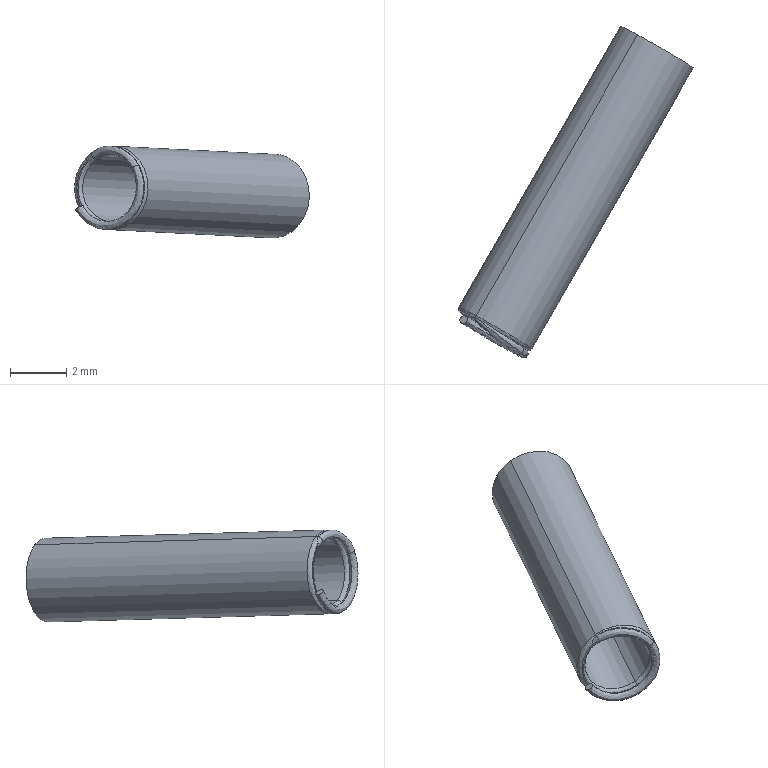Component | SolidWorks | ur3_15-0710z0-123-1 | 1 solid | 18 faces | box 8.38 x 11.84 x 3.29 mm | volume 30 mm3 | spline 11 | cylinder 4 | plane 3 | commonest cylinder face diameters 3 x2 2.4 x2
STEP:
#1=COLOUR_RGB('',0.7922,0.8196,0.9333);
#2=FILL_AREA_STYLE_COLOUR('',#1);
#3=FILL_AREA_STYLE('',(#2));
#4=SURFACE_STYLE_FILL_AREA(#3);
#5=SURFACE_SIDE_STYLE('',(#4));
#6=SURFACE_STYLE_USAGE(.BOTH.,#5);
#7=PRESENTATION_STYLE_ASSIGNMENT((#6));
#8=CARTESIAN_POINT('',(-3.463,-3.815,3.274));
#9=VERTEX_POINT('',#8);
#10=CARTESIAN_POINT('',(-3.409,-3.849,3.175));
#11=VERTEX_POINT('',#10);
#12=CARTESIAN_POINT('',(-3.436,-3.832,3.225));
#13=DIRECTION('',(0.4977,0.867,-0.02519));
#14=DIRECTION('',(-0.4585,0.2877,0.8408));
#15=AXIS2_PLACEMENT_3D('',#12,#13,#14);
#16=CIRCLE('',#15,0.05906);
#17=EDGE_CURVE('',#9,#11,#16,.T.);
#18=ORIENTED_EDGE('',*,*,#17,.F.);
#19=CARTESIAN_POINT('',(-3.464,-3.818,3.274));
#20=VERTEX_POINT('',#19);
#21=CARTESIAN_POINT('',(-3.461,-3.817,3.27));
#22=DIRECTION('',(0.7362,-0.4069,0.5407));
#23=DIRECTION('',(-0.4585,0.2877,0.8408));
#24=AXIS2_PLACEMENT_3D('',#21,#22,#23);
#25=CIRCLE('',#24,0.005906);
#26=EDGE_CURVE('',#9,#20,#25,.T.);
#27=ORIENTED_EDGE('',*,*,#26,.T.);
#28=CARTESIAN_POINT('',(-3.463,-3.819,3.275));
#29=VERTEX_POINT('',#28);
#30=CARTESIAN_POINT('',(-3.464,-3.818,3.274));
#31=CARTESIAN_POINT('',(-3.464,-3.819,3.274));
#32=CARTESIAN_POINT('',(-3.464,-3.819,3.274));
#33=CARTESIAN_POINT('',(-3.463,-3.819,3.275));
#34=B_SPLINE_CURVE_WITH_KNOTS('',3,(#30,#31,#32,#33),.UNSPECIFIED.,.F.,.F.,(4,4),(0.0003544,0.0003919),.UNSPECIFIED.);
#35=EDGE_CURVE('',#20,#29,#34,.T.);
#36=ORIENTED_EDGE('',*,*,#35,.T.);
#37=CARTESIAN_POINT('',(-3.461,-3.82,3.276));
#38=VERTEX_POINT('',#37);
#39=CARTESIAN_POINT('',(-3.463,-3.819,3.275));
#40=CARTESIAN_POINT('',(-3.463,-3.819,3.275));
#41=CARTESIAN_POINT('',(-3.462,-3.82,3.276));
#42=CARTESIAN_POINT('',(-3.461,-3.82,3.276));
#43=B_SPLINE_CURVE_WITH_KNOTS('',3,(#39,#40,#41,#42),.UNSPECIFIED.,.F.,.F.,(4,4),(0.0003919,0.0004641),.UNSPECIFIED.);
#44=EDGE_CURVE('',#29,#38,#43,.T.);
#45=ORIENTED_EDGE('',*,*,#44,.T.);
#46=CARTESIAN_POINT('',(-3.399,-3.86,3.255));
#47=VERTEX_POINT('',#46);
#48=CARTESIAN_POINT('',(-3.461,-3.82,3.276));
#49=CARTESIAN_POINT('',(-3.456,-3.823,3.28));
#50=CARTESIAN_POINT('',(-3.45,-3.826,3.282));
#51=CARTESIAN_POINT('',(-3.438,-3.834,3.283));
#52=CARTESIAN_POINT('',(-3.432,-3.838,3.282));
#53=CARTESIAN_POINT('',(-3.423,-3.844,3.279));
#54=CARTESIAN_POINT('',(-3.421,-3.845,3.278));
#55=CARTESIAN_POINT('',(-3.415,-3.849,3.275));
#56=CARTESIAN_POINT('',(-3.413,-3.85,3.273));
#57=CARTESIAN_POINT('',(-3.406,-3.855,3.266));
#58=CARTESIAN_POINT('',(-3.402,-3.858,3.261));
#59=CARTESIAN_POINT('',(-3.399,-3.86,3.255));
#60=B_SPLINE_CURVE_WITH_KNOTS('',3,(#48,#49,#50,#51,#52,#53,#54,#55,#56,#57,#58,#59),.UNSPECIFIED.,.F.,.F.,(4,2,2,2,2,4),(0.0004641,0.001005,0.001546,0.001817,0.002088,0.002629),.UNSPECIFIED.);
#61=EDGE_CURVE('',#38,#47,#60,.T.);
#62=ORIENTED_EDGE('',*,*,#61,.T.);
#63=CARTESIAN_POINT('',(-3.414,-3.853,3.179));
#64=VERTEX_POINT('',#63);
#65=CARTESIAN_POINT('',(-3.439,-3.837,3.225));
#66=DIRECTION('',(0.4977,0.867,-0.02519));
#67=DIRECTION('',(0.4585,-0.2877,-0.8408));
#68=AXIS2_PLACEMENT_3D('',#65,#66,#67);
#69=CIRCLE('',#68,0.05466);
#70=EDGE_CURVE('',#47,#64,#69,.T.);
#71=ORIENTED_EDGE('',*,*,#70,.T.);
#72=CARTESIAN_POINT('',(-3.412,-3.848,3.18));
#73=DIRECTION('',(-0.7362,0.4069,-0.5407));
#74=DIRECTION('',(0.4585,-0.2877,-0.8408));
#75=AXIS2_PLACEMENT_3D('',#72,#73,#74);
#76=CIRCLE('',#75,0.005906);
#77=EDGE_CURVE('',#11,#64,#76,.T.);
#78=ORIENTED_EDGE('',*,*,#77,.F.);
#79=EDGE_LOOP('',(#18,#27,#36,#45,#62,#71,#78));
#80=FACE_OUTER_BOUND('',#79,.T.);
#81=CARTESIAN_POINT('',(-3.463,-3.815,3.274));
#82=CARTESIAN_POINT('',(-3.376,-3.864,3.338));
#83=CARTESIAN_POINT('',(-3.322,-3.897,3.239));
#84=CARTESIAN_POINT('',(-3.409,-3.849,3.175));
#85=CARTESIAN_POINT('',(-3.465,-3.818,3.275));
#86=CARTESIAN_POINT('',(-3.378,-3.866,3.338));
#87=CARTESIAN_POINT('',(-3.324,-3.9,3.239));
#88=CARTESIAN_POINT('',(-3.411,-3.852,3.175));
#89=CARTESIAN_POINT('',(-3.465,-3.82,3.273));
#90=CARTESIAN_POINT('',(-3.381,-3.867,3.335));
#91=CARTESIAN_POINT('',(-3.328,-3.9,3.239));
#92=CARTESIAN_POINT('',(-3.412,-3.853,3.177));
#93=CARTESIAN_POINT('',(-3.464,-3.822,3.271));
#94=CARTESIAN_POINT('',(-3.384,-3.866,3.33));
#95=CARTESIAN_POINT('',(-3.334,-3.898,3.238));
#96=CARTESIAN_POINT('',(-3.414,-3.853,3.179));
#97=(BOUNDED_SURFACE()B_SPLINE_SURFACE(3,3,((#81,#82,#83,#84),(#85,#86,#87,#88),(#89,#90,#91,#92),(#93,#94,#95,#96)),.UNSPECIFIED.,.F.,.F.,.T.)B_SPLINE_SURFACE_WITH_KNOTS((4,4),(4,4),(0.,1.),(0.,1.),.UNSPECIFIED.)GEOMETRIC_REPRESENTATION_ITEM()RATIONAL_B_SPLINE_SURFACE(((1.,0.3333,0.3333,1.),(0.8617,0.2872,0.2872,0.8617),(0.8617,0.2872,0.2872,0.8617),(1.,0.3333,0.3333,1.)))REPRESENTATION_ITEM('')SURFACE());
#98=ADVANCED_FACE('',(#80),#97,.T.);
#99=CARTESIAN_POINT('',(-3.463,-3.822,3.27));
#100=VERTEX_POINT('',#99);
#101=CARTESIAN_POINT('',(-3.415,-3.852,3.18));
#102=VERTEX_POINT('',#101);
#103=CARTESIAN_POINT('',(-3.439,-3.837,3.225));
#104=DIRECTION('',(0.4977,0.867,-0.02519));
#105=DIRECTION('',(-0.4585,0.2877,0.8408));
#106=AXIS2_PLACEMENT_3D('',#103,#104,#105);
#107=CIRCLE('',#106,0.05315);
#108=EDGE_CURVE('',#100,#102,#107,.T.);
#109=ORIENTED_EDGE('',*,*,#108,.F.);
#110=CARTESIAN_POINT('',(-3.458,-3.818,3.265));
#111=VERTEX_POINT('',#110);
#112=CARTESIAN_POINT('',(-3.46,-3.817,3.27));
#113=DIRECTION('',(0.7362,-0.4069,0.5407));
#114=DIRECTION('',(-0.4585,0.2877,0.8408));
#115=AXIS2_PLACEMENT_3D('',#112,#113,#114);
#116=CIRCLE('',#115,0.005906);
#117=EDGE_CURVE('',#100,#111,#116,.T.);
#118=ORIENTED_EDGE('',*,*,#117,.T.);
#119=CARTESIAN_POINT('',(-3.414,-3.846,3.185));
#120=VERTEX_POINT('',#119);
#121=CARTESIAN_POINT('',(-3.436,-3.832,3.225));
#122=DIRECTION('',(0.4977,0.867,-0.02519));
#123=DIRECTION('',(0.4585,-0.2877,-0.8408));
#124=AXIS2_PLACEMENT_3D('',#121,#122,#123);
#125=CIRCLE('',#124,0.04724);
#126=EDGE_CURVE('',#111,#120,#125,.T.);
#127=ORIENTED_EDGE('',*,*,#126,.T.);
#128=CARTESIAN_POINT('',(-3.412,-3.847,3.18));
#129=DIRECTION('',(-0.7362,0.4069,-0.5407));
#130=DIRECTION('',(0.4585,-0.2877,-0.8408));
#131=AXIS2_PLACEMENT_3D('',#128,#129,#130);
#132=CIRCLE('',#131,0.005906);
#133=EDGE_CURVE('',#102,#120,#132,.T.);
#134=ORIENTED_EDGE('',*,*,#133,.F.);
#135=EDGE_LOOP('',(#109,#118,#127,#134));
#136=FACE_OUTER_BOUND('',#135,.T.);
#137=CARTESIAN_POINT('',(-3.463,-3.822,3.27));
#138=CARTESIAN_POINT('',(-3.385,-3.865,3.327));
#139=CARTESIAN_POINT('',(-3.336,-3.896,3.238));
#140=CARTESIAN_POINT('',(-3.415,-3.852,3.18));
#141=CARTESIAN_POINT('',(-3.462,-3.823,3.267));
#142=CARTESIAN_POINT('',(-3.389,-3.863,3.32));
#143=CARTESIAN_POINT('',(-3.343,-3.892,3.237));
#144=CARTESIAN_POINT('',(-3.416,-3.852,3.183));
#145=CARTESIAN_POINT('',(-3.459,-3.821,3.265));
#146=CARTESIAN_POINT('',(-3.39,-3.86,3.316));
#147=CARTESIAN_POINT('',(-3.347,-3.887,3.236));
#148=CARTESIAN_POINT('',(-3.416,-3.849,3.185));
#149=CARTESIAN_POINT('',(-3.458,-3.818,3.265));
#150=CARTESIAN_POINT('',(-3.388,-3.857,3.316));
#151=CARTESIAN_POINT('',(-3.345,-3.884,3.236));
#152=CARTESIAN_POINT('',(-3.414,-3.846,3.185));
#153=(BOUNDED_SURFACE()B_SPLINE_SURFACE(3,3,((#137,#138,#139,#140),(#141,#142,#143,#144),(#145,#146,#147,#148),(#149,#150,#151,#152)),.UNSPECIFIED.,.F.,.F.,.T.)B_SPLINE_SURFACE_WITH_KNOTS((4,4),(4,4),(0.,1.),(0.,1.),.UNSPECIFIED.)GEOMETRIC_REPRESENTATION_ITEM()RATIONAL_B_SPLINE_SURFACE(((1.,0.3333,0.3333,1.),(0.8047,0.2682,0.2682,0.8047),(0.8047,0.2682,0.2682,0.8047),(1.,0.3333,0.3333,1.)))REPRESENTATION_ITEM('')SURFACE());
#154=ADVANCED_FACE('',(#136),#153,.T.);
#155=ORIENTED_EDGE('',*,*,#108,.T.);
#156=CARTESIAN_POINT('',(-3.42,-3.856,3.185));
#157=VERTEX_POINT('',#156);
#158=CARTESIAN_POINT('',(-3.418,-3.858,3.18));
#159=DIRECTION('',(0.7362,-0.4069,0.5407));
#160=DIRECTION('',(0.4585,-0.2877,-0.8408));
#161=AXIS2_PLACEMENT_3D('',#158,#159,#160);
#162=CIRCLE('',#161,0.005906);
#163=EDGE_CURVE('',#102,#157,#162,.T.);
#164=ORIENTED_EDGE('',*,*,#163,.T.);
#165=CARTESIAN_POINT('',(-3.407,-3.862,3.251));
#166=VERTEX_POINT('',#165);
#167=CARTESIAN_POINT('',(-3.442,-3.842,3.225));
#168=DIRECTION('',(-0.4977,-0.867,0.02519));
#169=DIRECTION('',(-0.4585,0.2877,0.8408));
#170=AXIS2_PLACEMENT_3D('',#167,#168,#169);
#171=CIRCLE('',#170,0.04724);
#172=EDGE_CURVE('',#157,#166,#171,.T.);
#173=ORIENTED_EDGE('',*,*,#172,.T.);
#174=CARTESIAN_POINT('',(-3.462,-3.825,3.267));
#175=VERTEX_POINT('',#174);
#176=CARTESIAN_POINT('',(-3.462,-3.825,3.267));
#177=CARTESIAN_POINT('',(-3.458,-3.828,3.269));
#178=CARTESIAN_POINT('',(-3.453,-3.831,3.271));
#179=CARTESIAN_POINT('',(-3.445,-3.837,3.273));
#180=CARTESIAN_POINT('',(-3.442,-3.839,3.273));
#181=CARTESIAN_POINT('',(-3.437,-3.842,3.272));
#182=CARTESIAN_POINT('',(-3.436,-3.843,3.272));
#183=CARTESIAN_POINT('',(-3.434,-3.844,3.272));
#184=CARTESIAN_POINT('',(-3.432,-3.845,3.271));
#185=CARTESIAN_POINT('',(-3.431,-3.846,3.271));
#186=CARTESIAN_POINT('',(-3.43,-3.846,3.271));
#187=CARTESIAN_POINT('',(-3.43,-3.847,3.271));
#188=CARTESIAN_POINT('',(-3.43,-3.847,3.271));
#189=CARTESIAN_POINT('',(-3.42,-3.853,3.267));
#190=CARTESIAN_POINT('',(-3.412,-3.858,3.26));
#191=CARTESIAN_POINT('',(-3.407,-3.862,3.251));
#192=B_SPLINE_CURVE_WITH_KNOTS('',3,(#176,#177,#178,#179,#180,#181,#182,#183,#184,#185,#186,#187,#188,#189,#190,#191),.UNSPECIFIED.,.F.,.F.,(4,2,2,2,1,1,2,2,4),(0.,0.25,0.375,0.4375,0.4687,0.4844,0.4922,0.5,1.),.UNSPECIFIED.);
#193=EDGE_CURVE('',#175,#166,#192,.T.);
#194=ORIENTED_EDGE('',*,*,#193,.F.);
#195=CARTESIAN_POINT('',(-3.462,-3.824,3.266));
#196=VERTEX_POINT('',#195);
#197=CARTESIAN_POINT('',(-3.462,-3.825,3.267));
#198=CARTESIAN_POINT('',(-3.462,-3.825,3.267));
#199=CARTESIAN_POINT('',(-3.462,-3.825,3.266));
#200=CARTESIAN_POINT('',(-3.462,-3.824,3.266));
#201=B_SPLINE_CURVE_WITH_KNOTS('',3,(#197,#198,#199,#200),.UNSPECIFIED.,.F.,.F.,(4,4),(-0.00001925,0.),.UNSPECIFIED.);
#202=EDGE_CURVE('',#175,#196,#201,.T.);
#203=ORIENTED_EDGE('',*,*,#202,.T.);
#204=CARTESIAN_POINT('',(-3.466,-3.827,3.27));
#205=DIRECTION('',(-0.7362,0.4069,-0.5407));
#206=DIRECTION('',(-0.4585,0.2877,0.8408));
#207=AXIS2_PLACEMENT_3D('',#204,#205,#206);
#208=CIRCLE('',#207,0.005906);
#209=EDGE_CURVE('',#100,#196,#208,.T.);
#210=ORIENTED_EDGE('',*,*,#209,.F.);
#211=EDGE_LOOP('',(#155,#164,#173,#194,#203,#210));
#212=FACE_OUTER_BOUND('',#211,.T.);
#213=CARTESIAN_POINT('',(-3.415,-3.852,3.18));
#214=CARTESIAN_POINT('',(-3.336,-3.896,3.238));
#215=CARTESIAN_POINT('',(-3.385,-3.865,3.327));
#216=CARTESIAN_POINT('',(-3.463,-3.822,3.27));
#217=CARTESIAN_POINT('',(-3.416,-3.852,3.183));
#218=CARTESIAN_POINT('',(-3.343,-3.892,3.237));
#219=CARTESIAN_POINT('',(-3.389,-3.863,3.32));
#220=CARTESIAN_POINT('',(-3.462,-3.823,3.267));
#221=CARTESIAN_POINT('',(-3.419,-3.853,3.185));
#222=CARTESIAN_POINT('',(-3.349,-3.891,3.236));
#223=CARTESIAN_POINT('',(-3.392,-3.864,3.316));
#224=CARTESIAN_POINT('',(-3.462,-3.826,3.265));
#225=CARTESIAN_POINT('',(-3.42,-3.856,3.185));
#226=CARTESIAN_POINT('',(-3.351,-3.894,3.236));
#227=CARTESIAN_POINT('',(-3.394,-3.867,3.316));
#228=CARTESIAN_POINT('',(-3.464,-3.829,3.265));
#229=(BOUNDED_SURFACE()B_SPLINE_SURFACE(3,3,((#213,#214,#215,#216),(#217,#218,#219,#220),(#221,#222,#223,#224),(#225,#226,#227,#228)),.UNSPECIFIED.,.F.,.F.,.F.)B_SPLINE_SURFACE_WITH_KNOTS((4,4),(4,4),(0.,1.),(0.,1.),.UNSPECIFIED.)GEOMETRIC_REPRESENTATION_ITEM()RATIONAL_B_SPLINE_SURFACE(((1.,0.3333,0.3333,1.),(0.8047,0.2682,0.2682,0.8047),(0.8047,0.2682,0.2682,0.8047),(1.,0.3333,0.3333,1.)))REPRESENTATION_ITEM('')SURFACE());
#230=ADVANCED_FACE('',(#212),#229,.T.);
#231=ORIENTED_EDGE('',*,*,#202,.F.);
#232=CARTESIAN_POINT('',(-3.46,-3.82,3.27));
#233=DIRECTION('',(-0.6386,0.5513,-0.5369));
#234=DIRECTION('',(-0.4585,0.2877,0.8408));
#235=AXIS2_PLACEMENT_3D('',#232,#233,#234);
#236=CIRCLE('',#235,0.005906);
#237=EDGE_CURVE('',#175,#29,#236,.T.);
#238=ORIENTED_EDGE('',*,*,#237,.T.);
#239=ORIENTED_EDGE('',*,*,#35,.F.);
#240=CARTESIAN_POINT('',(-3.472,-3.818,3.262));
#241=VERTEX_POINT('',#240);
#242=CARTESIAN_POINT('',(-3.472,-3.818,3.262));
#243=CARTESIAN_POINT('',(-3.471,-3.818,3.265));
#244=CARTESIAN_POINT('',(-3.471,-3.818,3.267));
#245=CARTESIAN_POINT('',(-3.468,-3.817,3.271));
#246=CARTESIAN_POINT('',(-3.466,-3.818,3.272));
#247=CARTESIAN_POINT('',(-3.464,-3.818,3.274));
#248=B_SPLINE_CURVE_WITH_KNOTS('',3,(#242,#243,#244,#245,#246,#247),.UNSPECIFIED.,.F.,.F.,(4,2,4),(0.,0.0001772,0.0003544),.UNSPECIFIED.);
#249=EDGE_CURVE('',#241,#20,#248,.T.);
#250=ORIENTED_EDGE('',*,*,#249,.F.);
#251=CARTESIAN_POINT('',(-3.47,-3.819,3.261));
#252=VERTEX_POINT('',#251);
#253=CARTESIAN_POINT('',(-3.472,-3.818,3.262));
#254=CARTESIAN_POINT('',(-3.472,-3.818,3.262));
#255=CARTESIAN_POINT('',(-3.472,-3.818,3.262));
#256=CARTESIAN_POINT('',(-3.472,-3.818,3.262));
#257=CARTESIAN_POINT('',(-3.472,-3.818,3.262));
#258=CARTESIAN_POINT('',(-3.471,-3.818,3.261));
#259=CARTESIAN_POINT('',(-3.471,-3.818,3.261));
#260=CARTESIAN_POINT('',(-3.471,-3.818,3.261));
#261=CARTESIAN_POINT('',(-3.471,-3.818,3.261));
#262=CARTESIAN_POINT('',(-3.471,-3.818,3.261));
#263=CARTESIAN_POINT('',(-3.471,-3.818,3.261));
#264=CARTESIAN_POINT('',(-3.471,-3.818,3.261));
#265=CARTESIAN_POINT('',(-3.471,-3.818,3.261));
#266=CARTESIAN_POINT('',(-3.471,-3.818,3.261));
#267=CARTESIAN_POINT('',(-3.471,-3.818,3.261));
#268=CARTESIAN_POINT('',(-3.471,-3.818,3.261));
#269=CARTESIAN_POINT('',(-3.471,-3.818,3.261));
#270=CARTESIAN_POINT('',(-3.47,-3.819,3.261));
#271=CARTESIAN_POINT('',(-3.47,-3.819,3.261));
#272=B_SPLINE_CURVE_WITH_KNOTS('',3,(#253,#254,#255,#256,#257,#258,#259,#260,#261,#262,#263,#264,#265,#266,#267,#268,#269,#270,#271),.UNSPECIFIED.,.F.,.F.,(4,3,3,3,3,3,4),(0.,0.00001387,0.00002795,0.00003692,0.00004593,0.00005728,0.00006314),.UNSPECIFIED.);
#273=EDGE_CURVE('',#241,#252,#272,.T.);
#274=ORIENTED_EDGE('',*,*,#273,.T.);
#275=CARTESIAN_POINT('',(-3.462,-3.824,3.266));
#276=CARTESIAN_POINT('',(-3.464,-3.823,3.265));
#277=CARTESIAN_POINT('',(-3.465,-3.822,3.265));
#278=CARTESIAN_POINT('',(-3.468,-3.821,3.263));
#279=CARTESIAN_POINT('',(-3.469,-3.82,3.261));
#280=CARTESIAN_POINT('',(-3.47,-3.819,3.261));
#281=B_SPLINE_CURVE_WITH_KNOTS('',3,(#275,#276,#277,#278,#279,#280),.UNSPECIFIED.,.F.,.F.,(4,2,4),(0.,0.0001469,0.0002937),.UNSPECIFIED.);
#282=EDGE_CURVE('',#196,#252,#281,.T.);
#283=ORIENTED_EDGE('',*,*,#282,.F.);
#284=EDGE_LOOP('',(#231,#238,#239,#250,#274,#283));
#285=FACE_OUTER_BOUND('',#284,.T.);
#286=CARTESIAN_POINT('',(-3.462,-3.825,3.267));
#287=CARTESIAN_POINT('',(-3.464,-3.823,3.264));
#288=CARTESIAN_POINT('',(-3.467,-3.82,3.262));
#289=CARTESIAN_POINT('',(-3.469,-3.819,3.259));
#290=CARTESIAN_POINT('',(-3.465,-3.826,3.27));
#291=CARTESIAN_POINT('',(-3.468,-3.823,3.267));
#292=CARTESIAN_POINT('',(-3.471,-3.821,3.265));
#293=CARTESIAN_POINT('',(-3.473,-3.819,3.261));
#294=CARTESIAN_POINT('',(-3.466,-3.823,3.274));
#295=CARTESIAN_POINT('',(-3.469,-3.82,3.271));
#296=CARTESIAN_POINT('',(-3.472,-3.818,3.268));
#297=CARTESIAN_POINT('',(-3.474,-3.816,3.265));
#298=CARTESIAN_POINT('',(-3.463,-3.819,3.275));
#299=CARTESIAN_POINT('',(-3.466,-3.816,3.272));
#300=CARTESIAN_POINT('',(-3.469,-3.814,3.269));
#301=CARTESIAN_POINT('',(-3.472,-3.811,3.265));
#302=(BOUNDED_SURFACE()B_SPLINE_SURFACE(3,3,((#286,#287,#288,#289),(#290,#291,#292,#293),(#294,#295,#296,#297),(#298,#299,#300,#301)),.UNSPECIFIED.,.F.,.F.,.T.)B_SPLINE_SURFACE_WITH_KNOTS((4,4),(4,4),(0.,1.),(0.,1.),.UNSPECIFIED.)GEOMETRIC_REPRESENTATION_ITEM()RATIONAL_B_SPLINE_SURFACE(((1.,0.9948,0.9948,1.),(0.6746,0.6711,0.6711,0.6746),(0.6746,0.6711,0.6711,0.6746),(1.,0.9948,0.9948,1.)))REPRESENTATION_ITEM('')SURFACE());
#303=ADVANCED_FACE('',(#285),#302,.T.);
#304=CARTESIAN_POINT('',(-3.183,-3.455,3.164));
#305=VERTEX_POINT('',#304);
#306=CARTESIAN_POINT('',(-3.237,-3.421,3.263));
#307=VERTEX_POINT('',#306);
#308=CARTESIAN_POINT('',(-3.21,-3.438,3.213));
#309=DIRECTION('',(0.4977,0.867,-0.02519));
#310=DIRECTION('',(-0.4585,0.2877,0.8408));
#311=AXIS2_PLACEMENT_3D('',#308,#309,#310);
#312=CIRCLE('',#311,0.05906);
#313=EDGE_CURVE('',#305,#307,#312,.T.);
#314=ORIENTED_EDGE('',*,*,#313,.F.);
#315=CARTESIAN_POINT('',(-3.271,-3.608,3.168));
#316=DIRECTION('',(-0.4977,-0.867,0.02519));
#317=VECTOR('',#316,39.37);
#318=LINE('',#315,#317);
#319=EDGE_CURVE('',#305,#11,#318,.T.);
#320=ORIENTED_EDGE('',*,*,#319,.T.);
#321=CARTESIAN_POINT('',(-3.436,-3.832,3.225));
#322=DIRECTION('',(0.4977,0.867,-0.02519));
#323=DIRECTION('',(-0.4585,0.2877,0.8408));
#324=AXIS2_PLACEMENT_3D('',#321,#322,#323);
#325=CIRCLE('',#324,0.05906);
#326=EDGE_CURVE('',#11,#9,#325,.T.);
#327=ORIENTED_EDGE('',*,*,#326,.T.);
#328=CARTESIAN_POINT('',(-3.325,-3.574,3.267));
#329=DIRECTION('',(-0.4977,-0.867,0.02519));
#330=VECTOR('',#329,39.37);
#331=LINE('',#328,#330);
#332=EDGE_CURVE('',#307,#9,#331,.T.);
#333=ORIENTED_EDGE('',*,*,#332,.F.);
#334=EDGE_LOOP('',(#314,#320,#327,#333));
#335=FACE_OUTER_BOUND('',#334,.T.);
#336=CARTESIAN_POINT('',(-3.298,-3.591,3.218));
#337=DIRECTION('',(-0.4977,-0.867,0.02519));
#338=DIRECTION('',(-0.4585,0.2877,0.8408));
#339=AXIS2_PLACEMENT_3D('',#336,#337,#338);
#340=CYLINDRICAL_SURFACE('',#339,0.05906);
#341=ADVANCED_FACE('',(#335),#340,.T.);
#342=ORIENTED_EDGE('',*,*,#237,.F.);
#343=ORIENTED_EDGE('',*,*,#193,.T.);
#344=CARTESIAN_POINT('',(-3.399,-3.867,3.257));
#345=VERTEX_POINT('',#344);
#346=CARTESIAN_POINT('',(-3.403,-3.864,3.254));
#347=DIRECTION('',(0.4585,-0.2877,-0.8408));
#348=DIRECTION('',(0.7362,-0.4069,0.5407));
#349=AXIS2_PLACEMENT_3D('',#346,#347,#348);
#350=CIRCLE('',#349,0.005906);
#351=EDGE_CURVE('',#345,#166,#350,.T.);
#352=ORIENTED_EDGE('',*,*,#351,.F.);
#353=CARTESIAN_POINT('',(-3.436,-3.835,3.226));
#354=DIRECTION('',(-0.618,-0.7831,-0.06909));
#355=DIRECTION('',(-0.4585,0.2877,0.8408));
#356=AXIS2_PLACEMENT_3D('',#353,#354,#355);
#357=CIRCLE('',#356,0.05825);
#358=EDGE_CURVE('',#345,#38,#357,.T.);
#359=ORIENTED_EDGE('',*,*,#358,.T.);
#360=ORIENTED_EDGE('',*,*,#44,.F.);
#361=EDGE_LOOP('',(#342,#343,#352,#359,#360));
#362=FACE_OUTER_BOUND('',#361,.T.);
#363=CARTESIAN_POINT('',(-3.407,-3.861,3.251));
#364=CARTESIAN_POINT('',(-3.42,-3.854,3.274));
#365=CARTESIAN_POINT('',(-3.441,-3.837,3.279));
#366=CARTESIAN_POINT('',(-3.458,-3.822,3.265));
#367=CARTESIAN_POINT('',(-3.412,-3.87,3.251));
#368=CARTESIAN_POINT('',(-3.425,-3.862,3.275));
#369=CARTESIAN_POINT('',(-3.447,-3.845,3.281));
#370=CARTESIAN_POINT('',(-3.465,-3.83,3.265));
#371=CARTESIAN_POINT('',(-3.405,-3.875,3.256));
#372=CARTESIAN_POINT('',(-3.421,-3.865,3.285));
#373=CARTESIAN_POINT('',(-3.447,-3.845,3.292));
#374=CARTESIAN_POINT('',(-3.469,-3.826,3.274));
#375=CARTESIAN_POINT('',(-3.399,-3.867,3.257));
#376=CARTESIAN_POINT('',(-3.415,-3.857,3.286));
#377=CARTESIAN_POINT('',(-3.441,-3.837,3.293));
#378=CARTESIAN_POINT('',(-3.463,-3.818,3.275));
#379=(BOUNDED_SURFACE()B_SPLINE_SURFACE(3,3,((#363,#364,#365,#366),(#367,#368,#369,#370),(#371,#372,#373,#374),(#375,#376,#377,#378)),.UNSPECIFIED.,.F.,.F.,.T.)B_SPLINE_SURFACE_WITH_KNOTS((4,4),(4,4),(0.,1.),(0.,1.),.UNSPECIFIED.)GEOMETRIC_REPRESENTATION_ITEM()RATIONAL_B_SPLINE_SURFACE(((1.,0.8047,0.8047,1.),(0.3855,0.3102,0.3102,0.3855),(0.3855,0.3102,0.3102,0.3855),(1.,0.8047,0.8047,1.)))REPRESENTATION_ITEM('')SURFACE());
#380=ADVANCED_FACE('',(#362),#379,.T.);
#381=ORIENTED_EDGE('',*,*,#163,.F.);
#382=CARTESIAN_POINT('',(-3.439,-3.837,3.225));
#383=DIRECTION('',(0.4977,0.867,-0.02519));
#384=DIRECTION('',(-0.4585,0.2877,0.8408));
#385=AXIS2_PLACEMENT_3D('',#382,#383,#384);
#386=CIRCLE('',#385,0.05315);
#387=EDGE_CURVE('',#102,#100,#386,.T.);
#388=ORIENTED_EDGE('',*,*,#387,.T.);
#389=ORIENTED_EDGE('',*,*,#209,.T.);
#390=ORIENTED_EDGE('',*,*,#282,.T.);
#391=CARTESIAN_POINT('',(-3.477,-3.817,3.197));
#392=VERTEX_POINT('',#391);
#393=CARTESIAN_POINT('',(-3.439,-3.838,3.225));
#394=DIRECTION('',(0.4977,0.867,-0.02519));
#395=DIRECTION('',(-0.4585,0.2877,0.8408));
#396=AXIS2_PLACEMENT_3D('',#393,#394,#395);
#397=CIRCLE('',#396,0.05103);
#398=EDGE_CURVE('',#392,#252,#397,.T.);
#399=ORIENTED_EDGE('',*,*,#398,.F.);
#400=CARTESIAN_POINT('',(-3.477,-3.823,3.2));
#401=VERTEX_POINT('',#400);
#402=CARTESIAN_POINT('',(-3.477,-3.823,3.2));
#403=CARTESIAN_POINT('',(-3.476,-3.823,3.2));
#404=CARTESIAN_POINT('',(-3.476,-3.822,3.199));
#405=CARTESIAN_POINT('',(-3.476,-3.821,3.199));
#406=CARTESIAN_POINT('',(-3.476,-3.821,3.199));
#407=CARTESIAN_POINT('',(-3.476,-3.82,3.199));
#408=CARTESIAN_POINT('',(-3.476,-3.819,3.199));
#409=CARTESIAN_POINT('',(-3.476,-3.819,3.199));
#410=CARTESIAN_POINT('',(-3.476,-3.818,3.198));
#411=CARTESIAN_POINT('',(-3.476,-3.818,3.198));
#412=CARTESIAN_POINT('',(-3.476,-3.817,3.198));
#413=CARTESIAN_POINT('',(-3.477,-3.817,3.198));
#414=CARTESIAN_POINT('',(-3.477,-3.817,3.197));
#415=B_SPLINE_CURVE_WITH_KNOTS('',3,(#402,#403,#404,#405,#406,#407,#408,#409,#410,#411,#412,#413,#414),.UNSPECIFIED.,.F.,.F.,(4,3,3,3,4),(0.,0.00005037,0.0001007,0.0001511,0.0001795),.UNSPECIFIED.);
#416=EDGE_CURVE('',#401,#392,#415,.T.);
#417=ORIENTED_EDGE('',*,*,#416,.F.);
#418=CARTESIAN_POINT('',(-3.442,-3.842,3.225));
#419=DIRECTION('',(-0.4977,-0.867,0.02519));
#420=DIRECTION('',(-0.4585,0.2877,0.8408));
#421=AXIS2_PLACEMENT_3D('',#418,#419,#420);
#422=CIRCLE('',#421,0.04724);
#423=EDGE_CURVE('',#401,#157,#422,.T.);
#424=ORIENTED_EDGE('',*,*,#423,.T.);
#425=EDGE_LOOP('',(#381,#388,#389,#390,#399,#417,#424));
#426=FACE_OUTER_BOUND('',#425,.T.);
#427=CARTESIAN_POINT('',(-3.463,-3.822,3.27));
#428=CARTESIAN_POINT('',(-3.542,-3.779,3.212));
#429=CARTESIAN_POINT('',(-3.493,-3.809,3.123));
#430=CARTESIAN_POINT('',(-3.415,-3.852,3.18));
#431=CARTESIAN_POINT('',(-3.462,-3.823,3.267));
#432=CARTESIAN_POINT('',(-3.535,-3.782,3.213));
#433=CARTESIAN_POINT('',(-3.489,-3.811,3.129));
#434=CARTESIAN_POINT('',(-3.416,-3.852,3.183));
#435=CARTESIAN_POINT('',(-3.462,-3.826,3.265));
#436=CARTESIAN_POINT('',(-3.531,-3.787,3.214));
#437=CARTESIAN_POINT('',(-3.488,-3.814,3.134));
#438=CARTESIAN_POINT('',(-3.419,-3.853,3.185));
#439=CARTESIAN_POINT('',(-3.464,-3.829,3.265));
#440=CARTESIAN_POINT('',(-3.533,-3.79,3.214));
#441=CARTESIAN_POINT('',(-3.49,-3.817,3.134));
#442=CARTESIAN_POINT('',(-3.42,-3.856,3.185));
#443=(BOUNDED_SURFACE()B_SPLINE_SURFACE(3,3,((#427,#428,#429,#430),(#431,#432,#433,#434),(#435,#436,#437,#438),(#439,#440,#441,#442)),.UNSPECIFIED.,.F.,.F.,.T.)B_SPLINE_SURFACE_WITH_KNOTS((4,4),(4,4),(0.,1.),(0.,1.),.UNSPECIFIED.)GEOMETRIC_REPRESENTATION_ITEM()RATIONAL_B_SPLINE_SURFACE(((1.,0.3333,0.3333,1.),(0.8047,0.2682,0.2682,0.8047),(0.8047,0.2682,0.2682,0.8047),(1.,0.3333,0.3333,1.)))REPRESENTATION_ITEM('')SURFACE());
#444=ADVANCED_FACE('',(#426),#443,.T.);
#445=ORIENTED_EDGE('',*,*,#423,.F.);
#446=CARTESIAN_POINT('',(-3.485,-3.818,3.193));
#447=VERTEX_POINT('',#446);
#448=CARTESIAN_POINT('',(-3.485,-3.818,3.193));
#449=CARTESIAN_POINT('',(-3.486,-3.819,3.193));
#450=CARTESIAN_POINT('',(-3.486,-3.819,3.193));
#451=CARTESIAN_POINT('',(-3.486,-3.82,3.193));
#452=CARTESIAN_POINT('',(-3.486,-3.821,3.194));
#453=CARTESIAN_POINT('',(-3.486,-3.821,3.194));
#454=CARTESIAN_POINT('',(-3.486,-3.822,3.194));
#455=CARTESIAN_POINT('',(-3.486,-3.823,3.194));
#456=CARTESIAN_POINT('',(-3.486,-3.823,3.194));
#457=CARTESIAN_POINT('',(-3.486,-3.824,3.195));
#458=CARTESIAN_POINT('',(-3.486,-3.824,3.195));
#459=CARTESIAN_POINT('',(-3.485,-3.825,3.195));
#460=CARTESIAN_POINT('',(-3.485,-3.825,3.196));
#461=CARTESIAN_POINT('',(-3.484,-3.826,3.196));
#462=CARTESIAN_POINT('',(-3.484,-3.826,3.197));
#463=CARTESIAN_POINT('',(-3.483,-3.826,3.197));
#464=CARTESIAN_POINT('',(-3.483,-3.826,3.197));
#465=CARTESIAN_POINT('',(-3.482,-3.826,3.198));
#466=CARTESIAN_POINT('',(-3.482,-3.826,3.198));
#467=CARTESIAN_POINT('',(-3.481,-3.826,3.198));
#468=CARTESIAN_POINT('',(-3.481,-3.826,3.199));
#469=CARTESIAN_POINT('',(-3.48,-3.826,3.199));
#470=CARTESIAN_POINT('',(-3.479,-3.826,3.199));
#471=CARTESIAN_POINT('',(-3.479,-3.825,3.199));
#472=CARTESIAN_POINT('',(-3.478,-3.825,3.199));
#473=CARTESIAN_POINT('',(-3.478,-3.825,3.199));
#474=CARTESIAN_POINT('',(-3.477,-3.824,3.2));
#475=CARTESIAN_POINT('',(-3.477,-3.824,3.2));
#476=CARTESIAN_POINT('',(-3.477,-3.823,3.2));
#477=CARTESIAN_POINT('',(-3.477,-3.823,3.2));
#478=CARTESIAN_POINT('',(-3.477,-3.823,3.2));
#479=B_SPLINE_CURVE_WITH_KNOTS('',3,(#448,#449,#450,#451,#452,#453,#454,#455,#456,#457,#458,#459,#460,#461,#462,#463,#464,#465,#466,#467,#468,#469,#470,#471,#472,#473,#474,#475,#476,#477,#478),.UNSPECIFIED.,.F.,.F.,(4,3,3,3,3,3,3,3,3,3,4),(-0.0004689,-0.0004185,-0.0003681,-0.0003178,-0.0002674,-0.000217,-0.0001667,-0.0001163,-0.00006595,-0.00001558,0.),.UNSPECIFIED.);
#480=EDGE_CURVE('',#447,#401,#479,.T.);
#481=ORIENTED_EDGE('',*,*,#480,.F.);
#482=CARTESIAN_POINT('',(-3.398,-3.866,3.257));
#483=VERTEX_POINT('',#482);
#484=CARTESIAN_POINT('',(-3.442,-3.842,3.225));
#485=DIRECTION('',(-0.4977,-0.867,0.02519));
#486=DIRECTION('',(-0.4585,0.2877,0.8408));
#487=AXIS2_PLACEMENT_3D('',#484,#485,#486);
#488=CIRCLE('',#487,0.05906);
#489=EDGE_CURVE('',#447,#483,#488,.T.);
#490=ORIENTED_EDGE('',*,*,#489,.T.);
#491=CARTESIAN_POINT('',(-3.403,-3.864,3.254));
#492=DIRECTION('',(0.4585,-0.2877,-0.8408));
#493=DIRECTION('',(0.7362,-0.4069,0.5407));
#494=AXIS2_PLACEMENT_3D('',#491,#492,#493);
#495=CIRCLE('',#494,0.005906);
#496=EDGE_CURVE('',#483,#345,#495,.T.);
#497=ORIENTED_EDGE('',*,*,#496,.T.);
#498=ORIENTED_EDGE('',*,*,#351,.T.);
#499=ORIENTED_EDGE('',*,*,#172,.F.);
#500=EDGE_LOOP('',(#445,#481,#490,#497,#498,#499));
#501=FACE_OUTER_BOUND('',#500,.T.);
#502=CARTESIAN_POINT('',(-3.477,-3.823,3.2));
#503=CARTESIAN_POINT('',(-3.433,-3.85,3.12));
#504=CARTESIAN_POINT('',(-3.364,-3.889,3.171));
#505=CARTESIAN_POINT('',(-3.407,-3.862,3.251));
#506=CARTESIAN_POINT('',(-3.483,-3.833,3.2));
#507=CARTESIAN_POINT('',(-3.439,-3.861,3.12));
#508=CARTESIAN_POINT('',(-3.37,-3.899,3.172));
#509=CARTESIAN_POINT('',(-3.413,-3.872,3.251));
#510=CARTESIAN_POINT('',(-3.491,-3.829,3.193));
#511=CARTESIAN_POINT('',(-3.437,-3.863,3.094));
#512=CARTESIAN_POINT('',(-3.35,-3.911,3.158));
#513=CARTESIAN_POINT('',(-3.404,-3.877,3.257));
#514=CARTESIAN_POINT('',(-3.485,-3.818,3.193));
#515=CARTESIAN_POINT('',(-3.431,-3.852,3.094));
#516=CARTESIAN_POINT('',(-3.344,-3.9,3.158));
#517=CARTESIAN_POINT('',(-3.398,-3.866,3.257));
#518=(BOUNDED_SURFACE()B_SPLINE_SURFACE(3,3,((#502,#503,#504,#505),(#506,#507,#508,#509),(#510,#511,#512,#513),(#514,#515,#516,#517)),.UNSPECIFIED.,.F.,.F.,.T.)B_SPLINE_SURFACE_WITH_KNOTS((4,4),(4,4),(0.,1.),(0.,1.),.UNSPECIFIED.)GEOMETRIC_REPRESENTATION_ITEM()RATIONAL_B_SPLINE_SURFACE(((1.,0.3333,0.3333,1.),(0.3333,0.1111,0.1111,0.3333),(0.3333,0.1111,0.1111,0.3333),(1.,0.3333,0.3333,1.)))REPRESENTATION_ITEM('')SURFACE());
#519=ADVANCED_FACE('',(#501),#518,.T.);
#520=CARTESIAN_POINT('',(-3.231,-3.424,3.253));
#521=VERTEX_POINT('',#520);
#522=CARTESIAN_POINT('',(-3.188,-3.451,3.174));
#523=VERTEX_POINT('',#522);
#524=CARTESIAN_POINT('',(-3.21,-3.438,3.213));
#525=DIRECTION('',(0.4977,0.867,-0.02519));
#526=DIRECTION('',(-0.4585,0.2877,0.8408));
#527=AXIS2_PLACEMENT_3D('',#524,#525,#526);
#528=CIRCLE('',#527,0.04724);
#529=EDGE_CURVE('',#521,#523,#528,.T.);
#530=ORIENTED_EDGE('',*,*,#529,.T.);
#531=CARTESIAN_POINT('',(-3.276,-3.605,3.178));
#532=DIRECTION('',(-0.4977,-0.867,0.02519));
#533=VECTOR('',#532,39.37);
#534=LINE('',#531,#533);
#535=EDGE_CURVE('',#523,#120,#534,.T.);
#536=ORIENTED_EDGE('',*,*,#535,.T.);
#537=ORIENTED_EDGE('',*,*,#126,.F.);
#538=CARTESIAN_POINT('',(-3.32,-3.578,3.258));
#539=DIRECTION('',(-0.4977,-0.867,0.02519));
#540=VECTOR('',#539,39.37);
#541=LINE('',#538,#540);
#542=EDGE_CURVE('',#521,#111,#541,.T.);
#543=ORIENTED_EDGE('',*,*,#542,.F.);
#544=EDGE_LOOP('',(#530,#536,#537,#543));
#545=FACE_OUTER_BOUND('',#544,.T.);
#546=CARTESIAN_POINT('',(-3.298,-3.591,3.218));
#547=DIRECTION('',(-0.4977,-0.867,0.02519));
#548=DIRECTION('',(-0.4585,0.2877,0.8408));
#549=AXIS2_PLACEMENT_3D('',#546,#547,#548);
#550=CYLINDRICAL_SURFACE('',#549,0.04724);
#551=ADVANCED_FACE('',(#545),#550,.F.);
#552=ORIENTED_EDGE('',*,*,#319,.F.);
#553=CARTESIAN_POINT('',(-3.21,-3.438,3.213));
#554=DIRECTION('',(0.4977,0.867,-0.02519));
#555=DIRECTION('',(-0.4585,0.2877,0.8408));
#556=AXIS2_PLACEMENT_3D('',#553,#554,#555);
#557=CIRCLE('',#556,0.05906);
#558=EDGE_CURVE('',#307,#305,#557,.T.);
#559=ORIENTED_EDGE('',*,*,#558,.F.);
#560=ORIENTED_EDGE('',*,*,#332,.T.);
#561=ORIENTED_EDGE('',*,*,#17,.T.);
#562=EDGE_LOOP('',(#552,#559,#560,#561));
#563=FACE_OUTER_BOUND('',#562,.T.);
#564=CARTESIAN_POINT('',(-3.298,-3.591,3.218));
#565=DIRECTION('',(-0.4977,-0.867,0.02519));
#566=DIRECTION('',(-0.4585,0.2877,0.8408));
#567=AXIS2_PLACEMENT_3D('',#564,#565,#566);
#568=CYLINDRICAL_SURFACE('',#567,0.05906);
#569=ADVANCED_FACE('',(#563),#568,.T.);
#570=ORIENTED_EDGE('',*,*,#26,.F.);
#571=ORIENTED_EDGE('',*,*,#326,.F.);
#572=ORIENTED_EDGE('',*,*,#77,.T.);
#573=CARTESIAN_POINT('',(-3.479,-3.815,3.195));
#574=VERTEX_POINT('',#573);
#575=CARTESIAN_POINT('',(-3.439,-3.837,3.225));
#576=DIRECTION('',(0.4977,0.867,-0.02519));
#577=DIRECTION('',(0.4585,-0.2877,-0.8408));
#578=AXIS2_PLACEMENT_3D('',#575,#576,#577);
#579=CIRCLE('',#578,0.05466);
#580=EDGE_CURVE('',#64,#574,#579,.T.);
#581=ORIENTED_EDGE('',*,*,#580,.T.);
#582=CARTESIAN_POINT('',(-3.478,-3.816,3.196));
#583=VERTEX_POINT('',#582);
#584=CARTESIAN_POINT('',(-3.479,-3.815,3.195));
#585=CARTESIAN_POINT('',(-3.479,-3.815,3.196));
#586=CARTESIAN_POINT('',(-3.479,-3.816,3.196));
#587=CARTESIAN_POINT('',(-3.478,-3.816,3.196));
#588=B_SPLINE_CURVE_WITH_KNOTS('',3,(#584,#585,#586,#587),.UNSPECIFIED.,.F.,.F.,(4,4),(0.,0.00003873),.UNSPECIFIED.);
#589=EDGE_CURVE('',#574,#583,#588,.T.);
#590=ORIENTED_EDGE('',*,*,#589,.T.);
#591=CARTESIAN_POINT('',(-3.478,-3.816,3.196));
#592=CARTESIAN_POINT('',(-3.49,-3.808,3.218));
#593=CARTESIAN_POINT('',(-3.488,-3.809,3.244));
#594=CARTESIAN_POINT('',(-3.472,-3.818,3.262));
#595=(BOUNDED_CURVE()B_SPLINE_CURVE(3,(#591,#592,#593,#594),.UNSPECIFIED.,.F.,.F.)B_SPLINE_CURVE_WITH_KNOTS((4,4),(0.,1.),.UNSPECIFIED.)CURVE()GEOMETRIC_REPRESENTATION_ITEM()RATIONAL_B_SPLINE_CURVE((1.,0.8538,0.8538,1.))REPRESENTATION_ITEM(''));
#596=EDGE_CURVE('',#583,#241,#595,.T.);
#597=ORIENTED_EDGE('',*,*,#596,.T.);
#598=ORIENTED_EDGE('',*,*,#249,.T.);
#599=EDGE_LOOP('',(#570,#571,#572,#581,#590,#597,#598));
#600=FACE_OUTER_BOUND('',#599,.T.);
#601=CARTESIAN_POINT('',(-3.409,-3.849,3.175));
#602=CARTESIAN_POINT('',(-3.496,-3.801,3.111));
#603=CARTESIAN_POINT('',(-3.55,-3.767,3.211));
#604=CARTESIAN_POINT('',(-3.463,-3.815,3.274));
#605=CARTESIAN_POINT('',(-3.411,-3.852,3.175));
#606=CARTESIAN_POINT('',(-3.498,-3.804,3.111));
#607=CARTESIAN_POINT('',(-3.552,-3.77,3.211));
#608=CARTESIAN_POINT('',(-3.465,-3.818,3.275));
#609=CARTESIAN_POINT('',(-3.413,-3.854,3.177));
#610=CARTESIAN_POINT('',(-3.497,-3.808,3.116));
#611=CARTESIAN_POINT('',(-3.548,-3.775,3.211));
#612=CARTESIAN_POINT('',(-3.465,-3.821,3.273));
#613=CARTESIAN_POINT('',(-3.415,-3.853,3.18));
#614=CARTESIAN_POINT('',(-3.493,-3.81,3.123));
#615=CARTESIAN_POINT('',(-3.542,-3.779,3.212));
#616=CARTESIAN_POINT('',(-3.464,-3.822,3.27));
#617=(BOUNDED_SURFACE()B_SPLINE_SURFACE(3,3,((#601,#602,#603,#604),(#605,#606,#607,#608),(#609,#610,#611,#612),(#613,#614,#615,#616)),.UNSPECIFIED.,.F.,.F.,.F.)B_SPLINE_SURFACE_WITH_KNOTS((4,4),(4,4),(0.,1.),(0.,1.),.UNSPECIFIED.)GEOMETRIC_REPRESENTATION_ITEM()RATIONAL_B_SPLINE_SURFACE(((1.,0.3333,0.3333,1.),(0.8047,0.2682,0.2682,0.8047),(0.8047,0.2682,0.2682,0.8047),(1.,0.3333,0.3333,1.)))REPRESENTATION_ITEM('')SURFACE());
#618=ADVANCED_FACE('',(#600),#617,.T.);
#619=ORIENTED_EDGE('',*,*,#358,.F.);
#620=ORIENTED_EDGE('',*,*,#496,.F.);
#621=CARTESIAN_POINT('',(-3.403,-3.864,3.254));
#622=DIRECTION('',(0.4585,-0.2877,-0.8408));
#623=DIRECTION('',(0.7362,-0.4069,0.5407));
#624=AXIS2_PLACEMENT_3D('',#621,#622,#623);
#625=CIRCLE('',#624,0.005906);
#626=EDGE_CURVE('',#47,#483,#625,.T.);
#627=ORIENTED_EDGE('',*,*,#626,.F.);
#628=ORIENTED_EDGE('',*,*,#61,.F.);
#629=EDGE_LOOP('',(#619,#620,#627,#628));
#630=FACE_OUTER_BOUND('',#629,.T.);
#631=CARTESIAN_POINT('',(-3.399,-3.867,3.257));
#632=CARTESIAN_POINT('',(-3.414,-3.858,3.285));
#633=CARTESIAN_POINT('',(-3.44,-3.838,3.293));
#634=CARTESIAN_POINT('',(-3.461,-3.82,3.276));
#635=CARTESIAN_POINT('',(-3.397,-3.865,3.257));
#636=CARTESIAN_POINT('',(-3.412,-3.855,3.285));
#637=CARTESIAN_POINT('',(-3.438,-3.836,3.293));
#638=CARTESIAN_POINT('',(-3.459,-3.817,3.276));
#639=CARTESIAN_POINT('',(-3.397,-3.862,3.256));
#640=CARTESIAN_POINT('',(-3.412,-3.852,3.283));
#641=CARTESIAN_POINT('',(-3.436,-3.834,3.29));
#642=CARTESIAN_POINT('',(-3.457,-3.816,3.274));
#643=CARTESIAN_POINT('',(-3.399,-3.86,3.254));
#644=CARTESIAN_POINT('',(-3.413,-3.851,3.28));
#645=CARTESIAN_POINT('',(-3.436,-3.833,3.287));
#646=CARTESIAN_POINT('',(-3.455,-3.816,3.272));
#647=(BOUNDED_SURFACE()B_SPLINE_SURFACE(3,3,((#631,#632,#633,#634),(#635,#636,#637,#638),(#639,#640,#641,#642),(#643,#644,#645,#646)),.UNSPECIFIED.,.F.,.F.,.T.)B_SPLINE_SURFACE_WITH_KNOTS((4,4),(4,4),(0.,1.),(0.,1.),.UNSPECIFIED.)GEOMETRIC_REPRESENTATION_ITEM()RATIONAL_B_SPLINE_SURFACE(((1.,0.8138,0.8138,1.),(0.8222,0.6691,0.6691,0.8222),(0.8222,0.6691,0.6691,0.8222),(1.,0.8138,0.8138,1.)))REPRESENTATION_ITEM('')SURFACE());
#648=ADVANCED_FACE('',(#630),#647,.T.);
#649=ORIENTED_EDGE('',*,*,#596,.F.);
#650=CARTESIAN_POINT('',(-3.459,-3.827,3.211));
#651=DIRECTION('',(0.7362,-0.4069,0.5407));
#652=VECTOR('',#651,39.37);
#653=LINE('',#650,#652);
#654=EDGE_CURVE('',#583,#392,#653,.T.);
#655=ORIENTED_EDGE('',*,*,#654,.T.);
#656=ORIENTED_EDGE('',*,*,#398,.T.);
#657=ORIENTED_EDGE('',*,*,#273,.F.);
#658=EDGE_LOOP('',(#649,#655,#656,#657));
#659=FACE_OUTER_BOUND('',#658,.T.);
#660=CARTESIAN_POINT('',(-3.459,-3.827,3.211));
#661=DIRECTION('',(-0.4977,-0.867,0.02519));
#662=DIRECTION('',(-0.7362,0.4069,-0.5407));
#663=AXIS2_PLACEMENT_3D('',#660,#661,#662);
#664=PLANE('',#663);
#665=ADVANCED_FACE('',(#659),#664,.T.);
#666=ORIENTED_EDGE('',*,*,#589,.F.);
#667=CARTESIAN_POINT('',(-3.479,-3.815,3.195));
#668=CARTESIAN_POINT('',(-3.48,-3.815,3.195));
#669=CARTESIAN_POINT('',(-3.48,-3.815,3.195));
#670=CARTESIAN_POINT('',(-3.481,-3.815,3.194));
#671=CARTESIAN_POINT('',(-3.482,-3.815,3.194));
#672=CARTESIAN_POINT('',(-3.482,-3.815,3.194));
#673=CARTESIAN_POINT('',(-3.483,-3.816,3.194));
#674=CARTESIAN_POINT('',(-3.483,-3.816,3.194));
#675=CARTESIAN_POINT('',(-3.484,-3.816,3.193));
#676=CARTESIAN_POINT('',(-3.484,-3.817,3.193));
#677=CARTESIAN_POINT('',(-3.485,-3.817,3.193));
#678=CARTESIAN_POINT('',(-3.485,-3.818,3.193));
#679=CARTESIAN_POINT('',(-3.485,-3.818,3.193));
#680=B_SPLINE_CURVE_WITH_KNOTS('',3,(#667,#668,#669,#670,#671,#672,#673,#674,#675,#676,#677,#678,#679),.UNSPECIFIED.,.F.,.F.,(4,3,3,3,4),(-0.0006646,-0.0006143,-0.0005639,-0.0005135,-0.0004689),.UNSPECIFIED.);
#681=EDGE_CURVE('',#574,#447,#680,.T.);
#682=ORIENTED_EDGE('',*,*,#681,.T.);
#683=ORIENTED_EDGE('',*,*,#480,.T.);
#684=ORIENTED_EDGE('',*,*,#416,.T.);
#685=ORIENTED_EDGE('',*,*,#654,.F.);
#686=EDGE_LOOP('',(#666,#682,#683,#684,#685));
#687=FACE_OUTER_BOUND('',#686,.T.);
#688=CARTESIAN_POINT('',(-3.481,-3.821,3.196));
#689=DIRECTION('',(-0.4585,0.2877,0.8408));
#690=DIRECTION('',(0.7362,-0.4069,0.5407));
#691=AXIS2_PLACEMENT_3D('',#688,#689,#690);
#692=PLANE('',#691);
#693=ADVANCED_FACE('',(#687),#692,.T.);
#694=ORIENTED_EDGE('',*,*,#489,.F.);
#695=ORIENTED_EDGE('',*,*,#681,.F.);
#696=ORIENTED_EDGE('',*,*,#580,.F.);
#697=ORIENTED_EDGE('',*,*,#70,.F.);
#698=ORIENTED_EDGE('',*,*,#626,.T.);
#699=EDGE_LOOP('',(#694,#695,#696,#697,#698));
#700=FACE_OUTER_BOUND('',#699,.T.);
#701=CARTESIAN_POINT('',(-3.485,-3.818,3.193));
#702=CARTESIAN_POINT('',(-3.431,-3.852,3.094));
#703=CARTESIAN_POINT('',(-3.344,-3.9,3.158));
#704=CARTESIAN_POINT('',(-3.398,-3.866,3.257));
#705=CARTESIAN_POINT('',(-3.484,-3.816,3.193));
#706=CARTESIAN_POINT('',(-3.43,-3.85,3.094));
#707=CARTESIAN_POINT('',(-3.343,-3.898,3.158));
#708=CARTESIAN_POINT('',(-3.397,-3.864,3.257));
#709=CARTESIAN_POINT('',(-3.482,-3.815,3.194));
#710=CARTESIAN_POINT('',(-3.429,-3.848,3.098));
#711=CARTESIAN_POINT('',(-3.345,-3.894,3.16));
#712=CARTESIAN_POINT('',(-3.397,-3.861,3.256));
#713=CARTESIAN_POINT('',(-3.479,-3.815,3.195));
#714=CARTESIAN_POINT('',(-3.429,-3.847,3.103));
#715=CARTESIAN_POINT('',(-3.349,-3.891,3.163));
#716=CARTESIAN_POINT('',(-3.399,-3.86,3.255));
#717=(BOUNDED_SURFACE()B_SPLINE_SURFACE(3,3,((#701,#702,#703,#704),(#705,#706,#707,#708),(#709,#710,#711,#712),(#713,#714,#715,#716)),.UNSPECIFIED.,.F.,.F.,.T.)B_SPLINE_SURFACE_WITH_KNOTS((4,4),(4,4),(0.,1.),(0.,1.),.UNSPECIFIED.)GEOMETRIC_REPRESENTATION_ITEM()RATIONAL_B_SPLINE_SURFACE(((1.,0.3333,0.3333,1.),(0.8617,0.2872,0.2872,0.8617),(0.8617,0.2872,0.2872,0.8617),(1.,0.3333,0.3333,1.)))REPRESENTATION_ITEM('')SURFACE());
#718=ADVANCED_FACE('',(#700),#717,.T.);
#719=ORIENTED_EDGE('',*,*,#117,.F.);
#720=ORIENTED_EDGE('',*,*,#387,.F.);
#721=ORIENTED_EDGE('',*,*,#133,.T.);
#722=CARTESIAN_POINT('',(-3.436,-3.832,3.225));
#723=DIRECTION('',(0.4977,0.867,-0.02519));
#724=DIRECTION('',(0.4585,-0.2877,-0.8408));
#725=AXIS2_PLACEMENT_3D('',#722,#723,#724);
#726=CIRCLE('',#725,0.04724);
#727=EDGE_CURVE('',#120,#111,#726,.T.);
#728=ORIENTED_EDGE('',*,*,#727,.T.);
#729=EDGE_LOOP('',(#719,#720,#721,#728));
#730=FACE_OUTER_BOUND('',#729,.T.);
#731=CARTESIAN_POINT('',(-3.415,-3.852,3.18));
#732=CARTESIAN_POINT('',(-3.493,-3.809,3.123));
#733=CARTESIAN_POINT('',(-3.542,-3.779,3.212));
#734=CARTESIAN_POINT('',(-3.463,-3.822,3.27));
#735=CARTESIAN_POINT('',(-3.416,-3.852,3.183));
#736=CARTESIAN_POINT('',(-3.489,-3.811,3.129));
#737=CARTESIAN_POINT('',(-3.535,-3.782,3.213));
#738=CARTESIAN_POINT('',(-3.462,-3.823,3.267));
#739=CARTESIAN_POINT('',(-3.416,-3.849,3.185));
#740=CARTESIAN_POINT('',(-3.486,-3.81,3.134));
#741=CARTESIAN_POINT('',(-3.529,-3.783,3.214));
#742=CARTESIAN_POINT('',(-3.459,-3.821,3.265));
#743=CARTESIAN_POINT('',(-3.414,-3.846,3.185));
#744=CARTESIAN_POINT('',(-3.484,-3.807,3.134));
#745=CARTESIAN_POINT('',(-3.527,-3.78,3.213));
#746=CARTESIAN_POINT('',(-3.458,-3.818,3.265));
#747=(BOUNDED_SURFACE()B_SPLINE_SURFACE(3,3,((#731,#732,#733,#734),(#735,#736,#737,#738),(#739,#740,#741,#742),(#743,#744,#745,#746)),.UNSPECIFIED.,.F.,.F.,.T.)B_SPLINE_SURFACE_WITH_KNOTS((4,4),(4,4),(0.,1.),(0.,1.),.UNSPECIFIED.)GEOMETRIC_REPRESENTATION_ITEM()RATIONAL_B_SPLINE_SURFACE(((1.,0.3333,0.3333,1.),(0.8047,0.2682,0.2682,0.8047),(0.8047,0.2682,0.2682,0.8047),(1.,0.3333,0.3333,1.)))REPRESENTATION_ITEM('')SURFACE());
#748=ADVANCED_FACE('',(#730),#747,.T.);
#749=ORIENTED_EDGE('',*,*,#535,.F.);
#750=CARTESIAN_POINT('',(-3.21,-3.438,3.213));
#751=DIRECTION('',(0.4977,0.867,-0.02519));
#752=DIRECTION('',(-0.4585,0.2877,0.8408));
#753=AXIS2_PLACEMENT_3D('',#750,#751,#752);
#754=CIRCLE('',#753,0.04724);
#755=EDGE_CURVE('',#523,#521,#754,.T.);
#756=ORIENTED_EDGE('',*,*,#755,.T.);
#757=ORIENTED_EDGE('',*,*,#542,.T.);
#758=ORIENTED_EDGE('',*,*,#727,.F.);
#759=EDGE_LOOP('',(#749,#756,#757,#758));
#760=FACE_OUTER_BOUND('',#759,.T.);
#761=CARTESIAN_POINT('',(-3.298,-3.591,3.218));
#762=DIRECTION('',(-0.4977,-0.867,0.02519));
#763=DIRECTION('',(-0.4585,0.2877,0.8408));
#764=AXIS2_PLACEMENT_3D('',#761,#762,#763);
#765=CYLINDRICAL_SURFACE('',#764,0.04724);
#766=ADVANCED_FACE('',(#760),#765,.F.);
#767=ORIENTED_EDGE('',*,*,#558,.T.);
#768=ORIENTED_EDGE('',*,*,#313,.T.);
#769=EDGE_LOOP('',(#767,#768));
#770=FACE_OUTER_BOUND('',#769,.T.);
#771=ORIENTED_EDGE('',*,*,#529,.F.);
#772=ORIENTED_EDGE('',*,*,#755,.F.);
#773=EDGE_LOOP('',(#771,#772));
#774=FACE_BOUND('',#773,.T.);
#775=CARTESIAN_POINT('',(-3.216,-3.421,3.672));
#776=DIRECTION('',(-0.4977,-0.867,0.02519));
#777=DIRECTION('',(-0.4585,0.2877,0.8408));
#778=AXIS2_PLACEMENT_3D('',#775,#776,#777);
#779=PLANE('',#778);
#780=ADVANCED_FACE('',(#770,#774),#779,.F.);
#781=CLOSED_SHELL('',(#98,#154,#230,#303,#341,#380,#444,#519,#551,#569,#618,#648,#665,#693,#718,#748,#766,#780));
#782=MANIFOLD_SOLID_BREP('',#781);
#783=STYLED_ITEM('',(#7),#782);
#784=PRESENTATION_LAYER_ASSIGNMENT('','',(#783));
#785=CARTESIAN_POINT('',(0.,0.,0.));
#786=DIRECTION('',(0.,0.,1.));
#787=DIRECTION('',(1.,0.,0.));
#788=AXIS2_PLACEMENT_3D('',#785,#786,#787);
#789=(LENGTH_UNIT()NAMED_UNIT(*)SI_UNIT($,.METRE.));
#790=LENGTH_MEASURE_WITH_UNIT(LENGTH_MEASURE(0.0254),#789);
#791=DIMENSIONAL_EXPONENTS(1.,0.,0.,0.,0.,0.,0.);
#792=(CONVERSION_BASED_UNIT('',#790)LENGTH_UNIT()NAMED_UNIT(#791));
#793=UNCERTAINTY_MEASURE_WITH_UNIT(LENGTH_MEASURE(0.00001),#792,'','');
#794=(NAMED_UNIT(*)PLANE_ANGLE_UNIT()SI_UNIT($,.RADIAN.));
#795=(NAMED_UNIT(*)SI_UNIT($,.STERADIAN.)SOLID_ANGLE_UNIT());
#796=(GEOMETRIC_REPRESENTATION_CONTEXT(3)GLOBAL_UNCERTAINTY_ASSIGNED_CONTEXT((#793))GLOBAL_UNIT_ASSIGNED_CONTEXT((#792,#794,#795))REPRESENTATION_CONTEXT('',''));
#797=ADVANCED_BREP_SHAPE_REPRESENTATION('',(#782,#788),#796);
#798=(LENGTH_UNIT()NAMED_UNIT(*)SI_UNIT($,.METRE.));
#799=LENGTH_MEASURE_WITH_UNIT(LENGTH_MEASURE(0.0254),#798);
#800=DIMENSIONAL_EXPONENTS(1.,0.,0.,0.,0.,0.,0.);
#801=(CONVERSION_BASED_UNIT('',#799)LENGTH_UNIT()NAMED_UNIT(#800));
#802=UNCERTAINTY_MEASURE_WITH_UNIT(LENGTH_MEASURE(0.00001),#801,'','');
#803=(NAMED_UNIT(*)PLANE_ANGLE_UNIT()SI_UNIT($,.RADIAN.));
#804=(NAMED_UNIT(*)SI_UNIT($,.STERADIAN.)SOLID_ANGLE_UNIT());
#805=(GEOMETRIC_REPRESENTATION_CONTEXT(3)GLOBAL_UNCERTAINTY_ASSIGNED_CONTEXT((#802))GLOBAL_UNIT_ASSIGNED_CONTEXT((#801,#803,#804))REPRESENTATION_CONTEXT('',''));
#806=MECHANICAL_DESIGN_GEOMETRIC_PRESENTATION_REPRESENTATION('',(#783),#805);